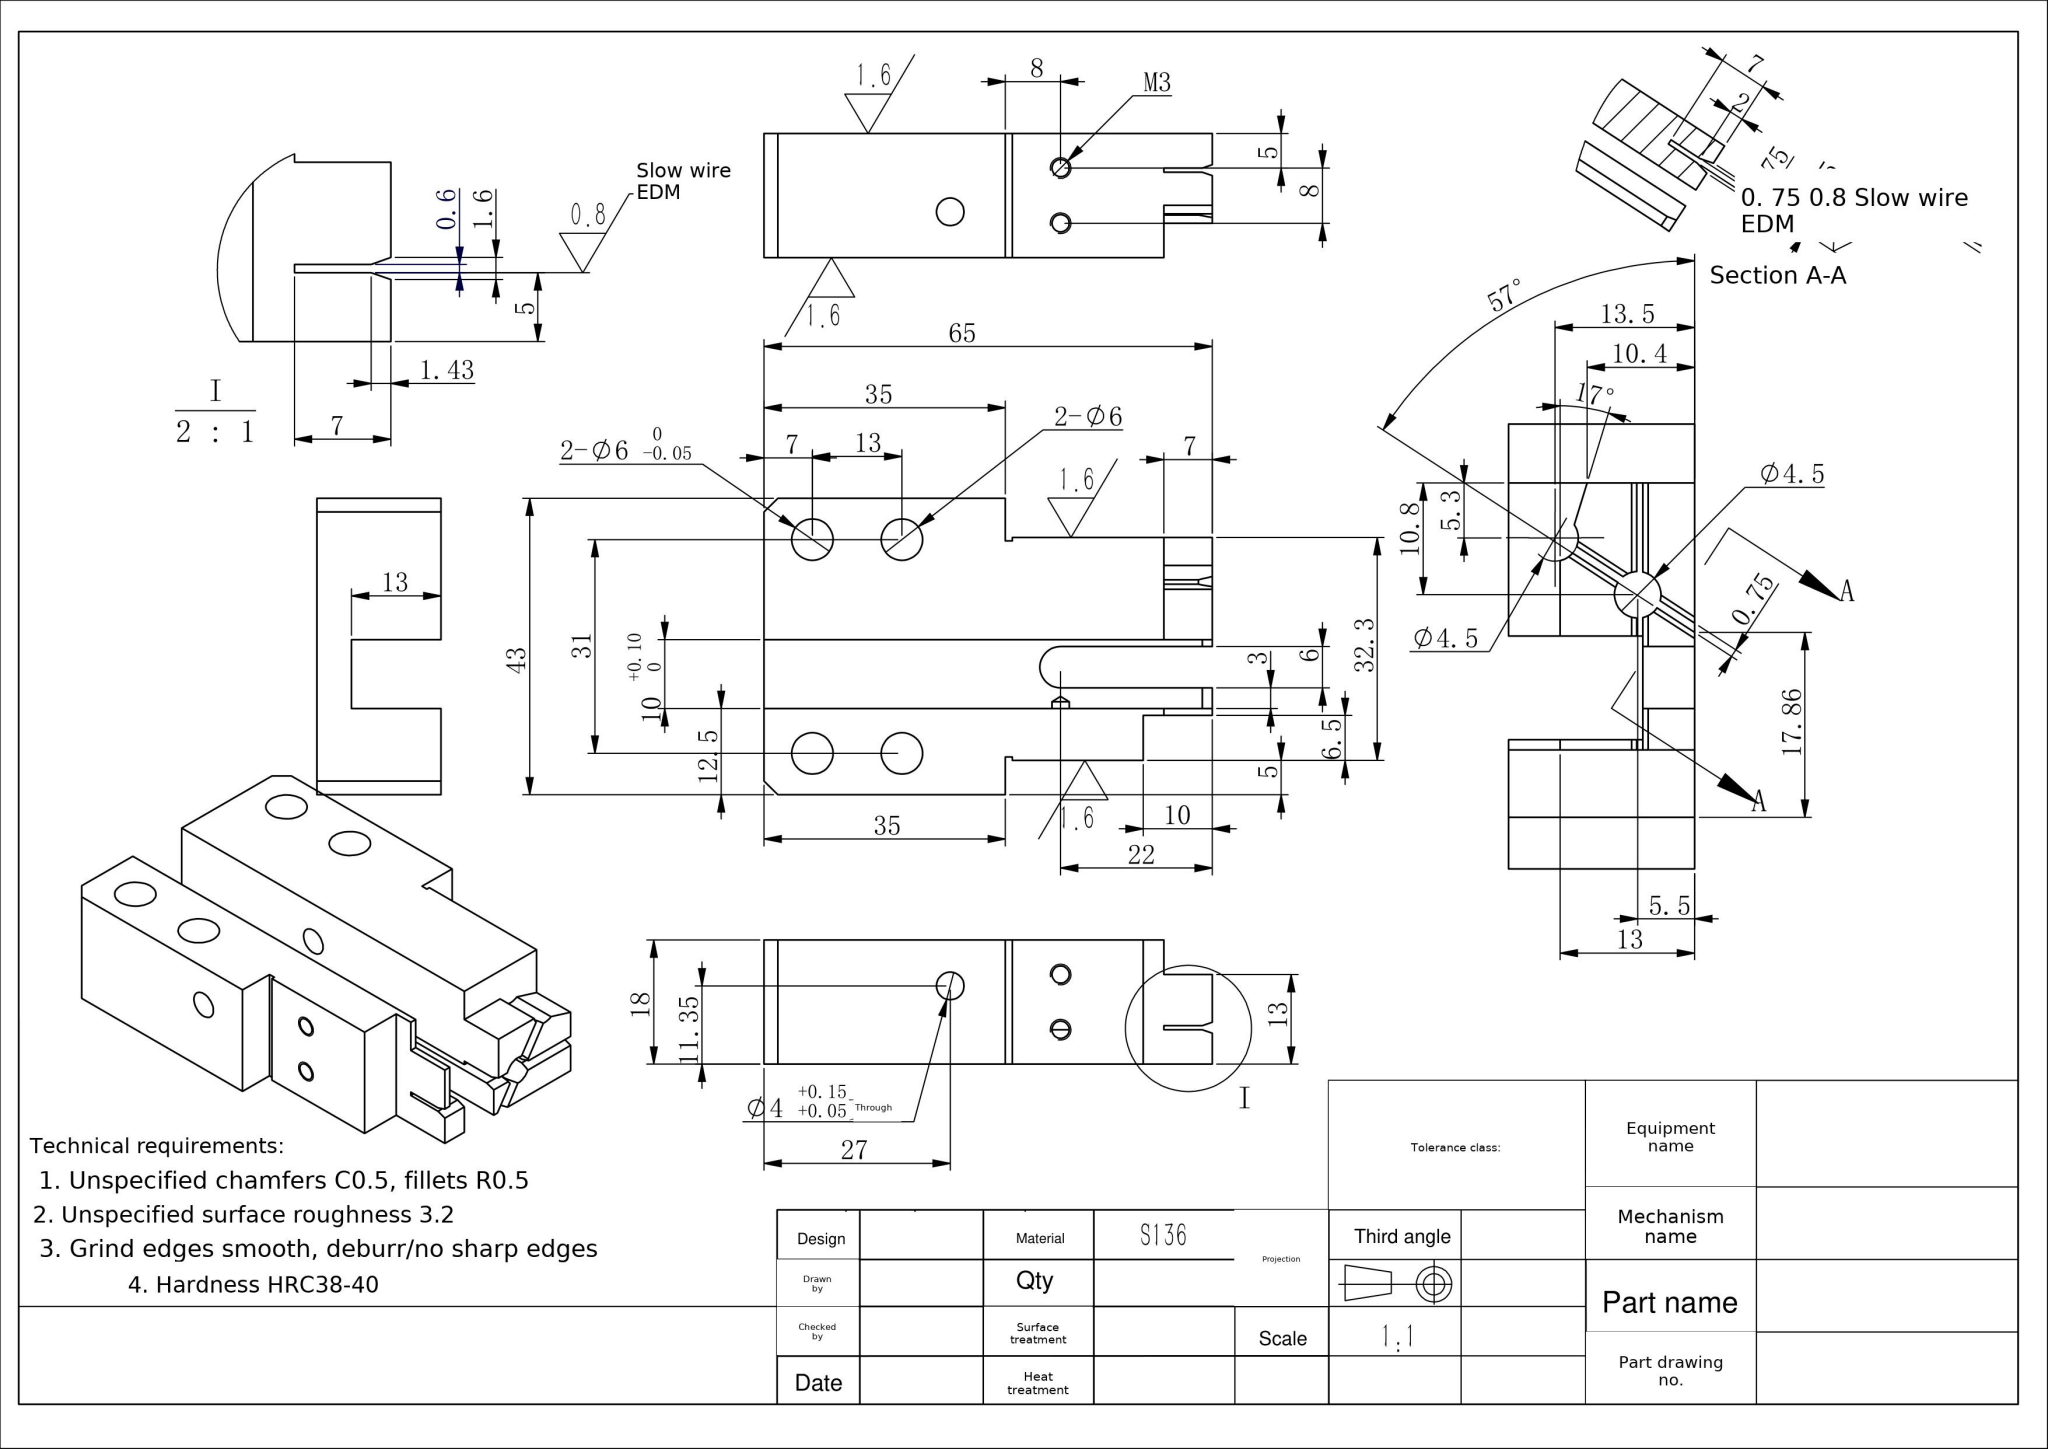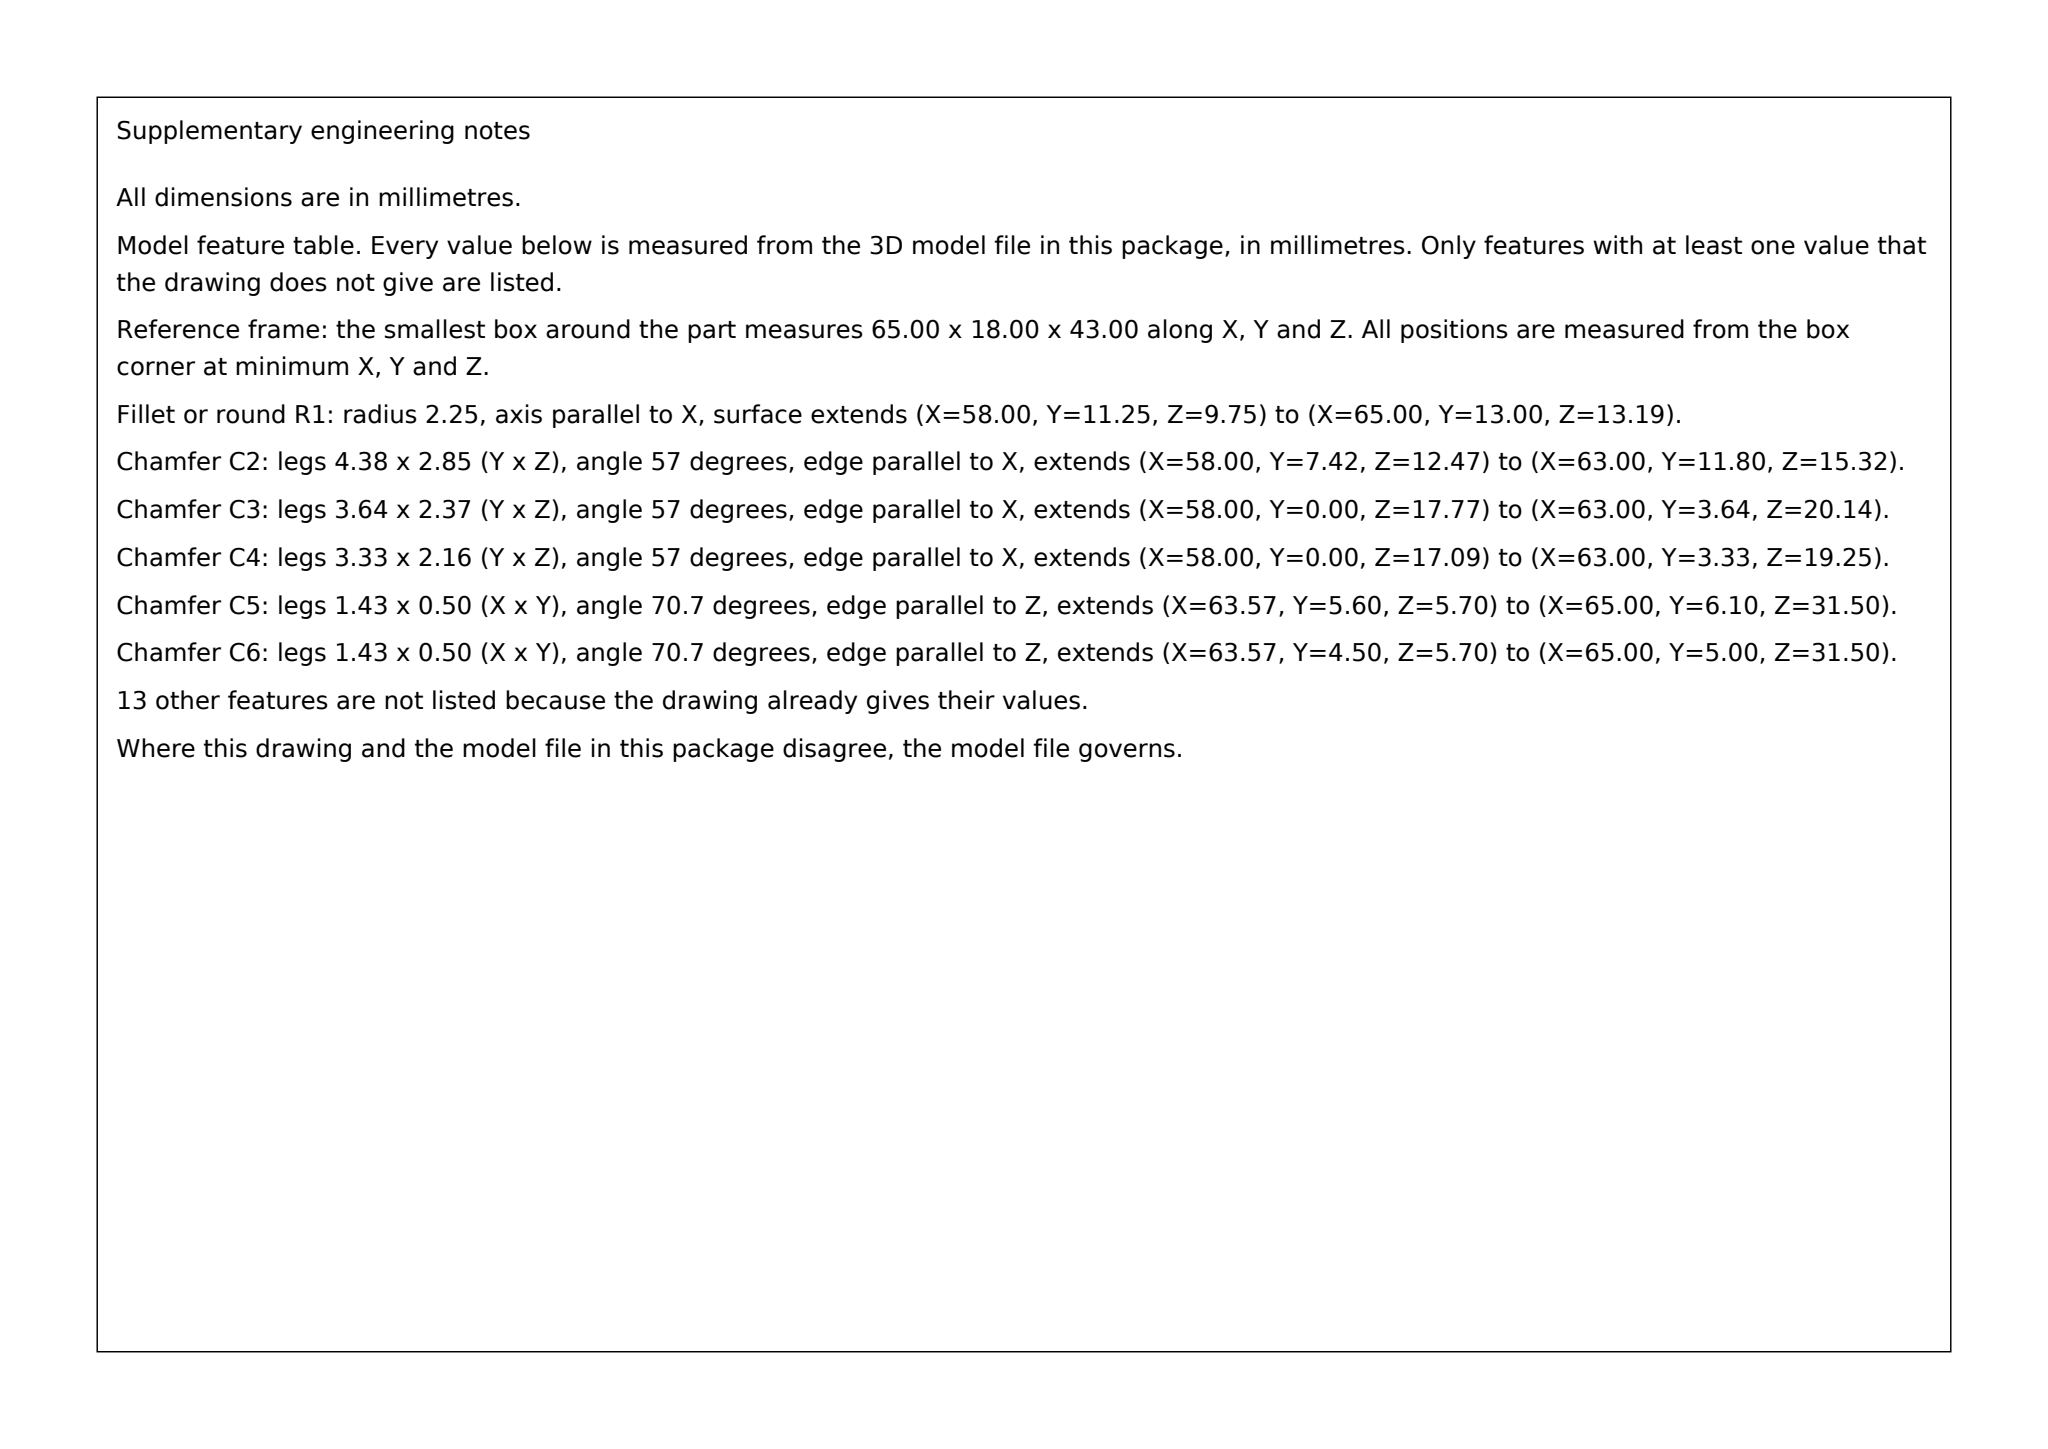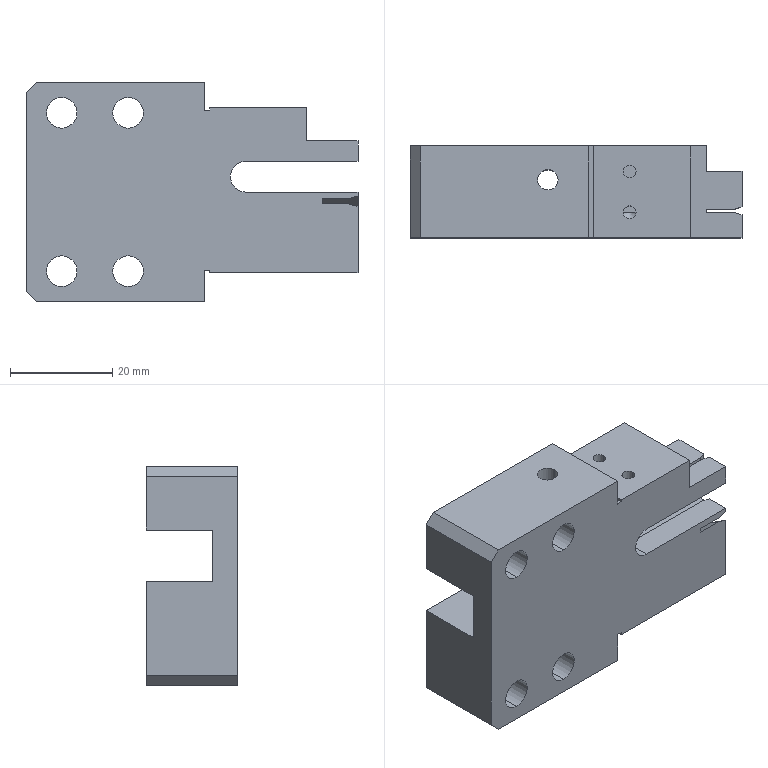Part | SolidWorks | mm | material S136 | 1 solid | 85 faces | box 65 x 18 x 43 mm | volume 30608 mm3 | plane 53 | cylinder 27 | cone 5 | commonest cylinder face diameters 6 x9 2.5 x8 4.5 x6 4 x4